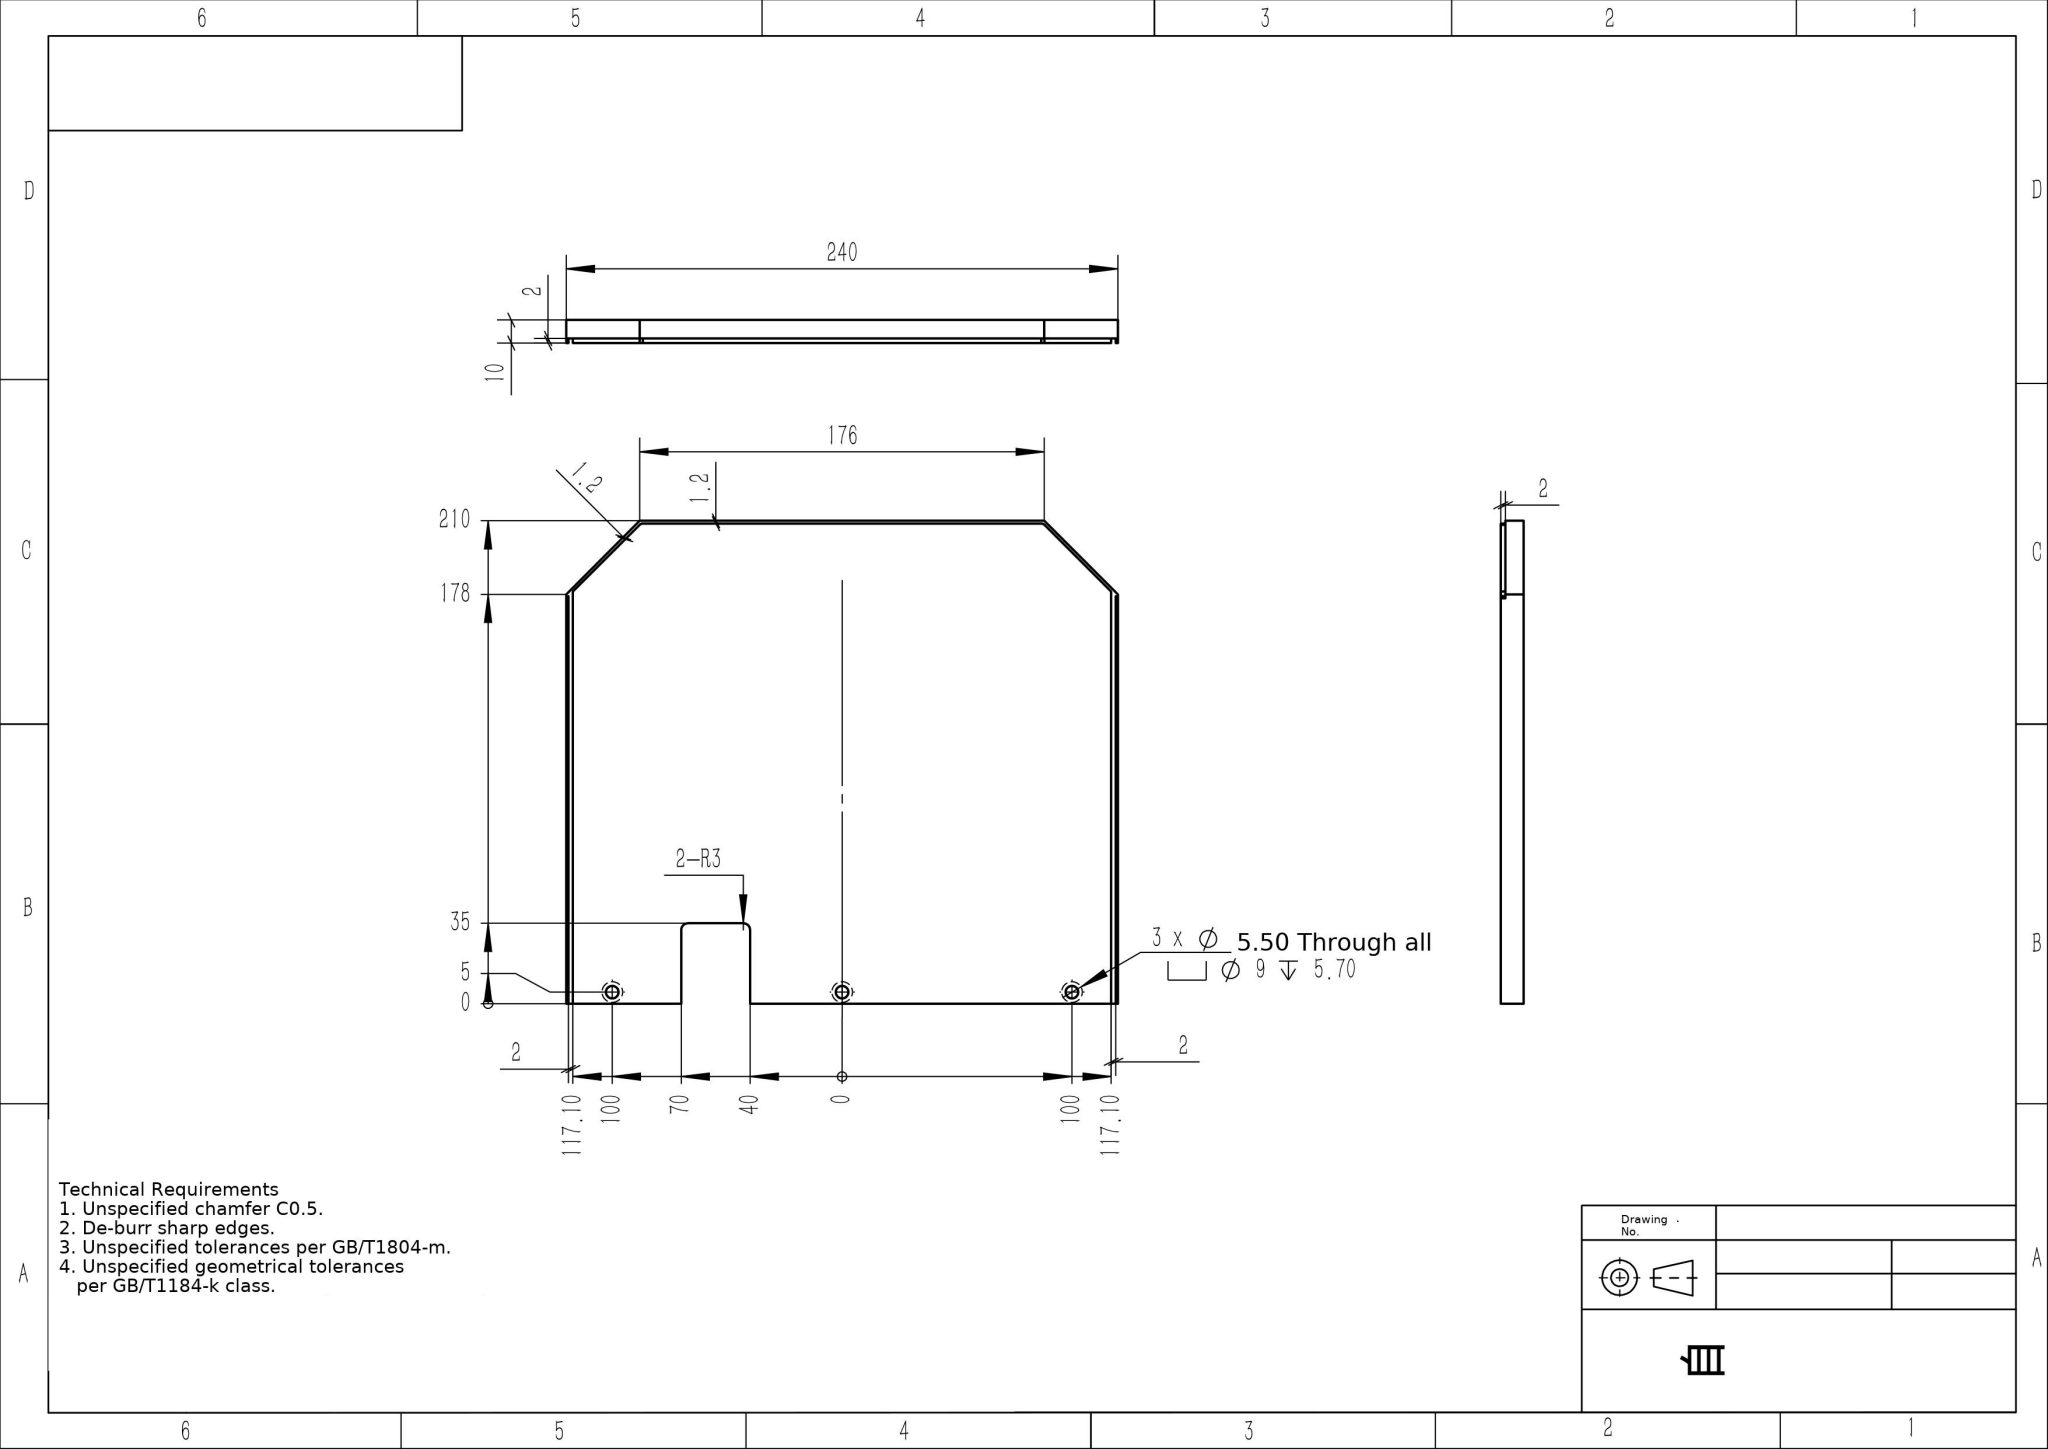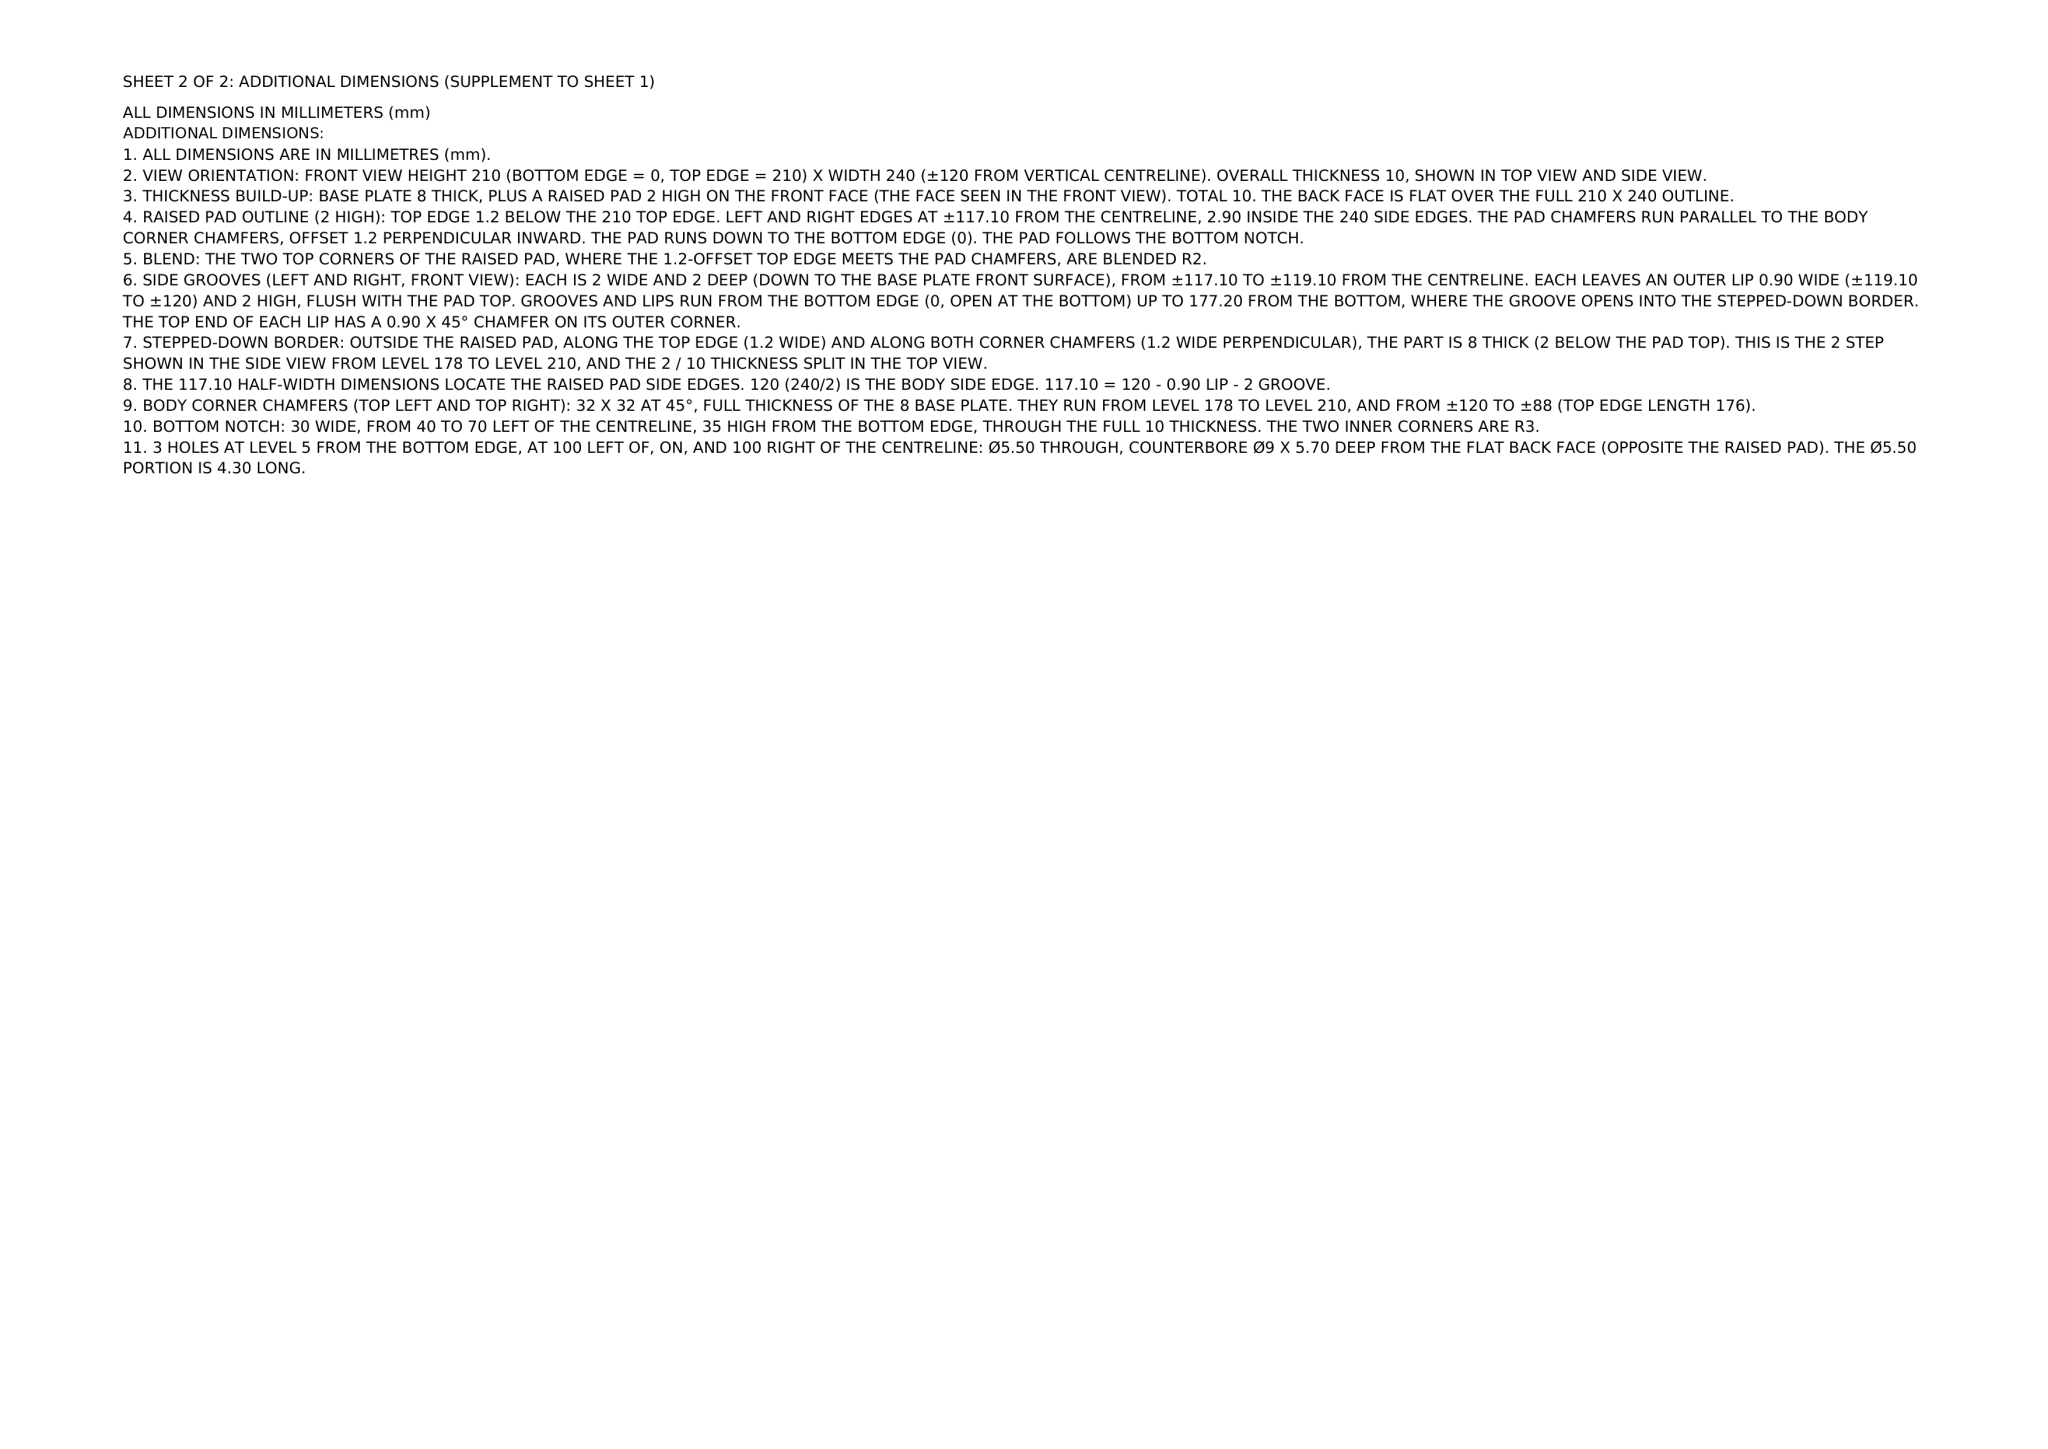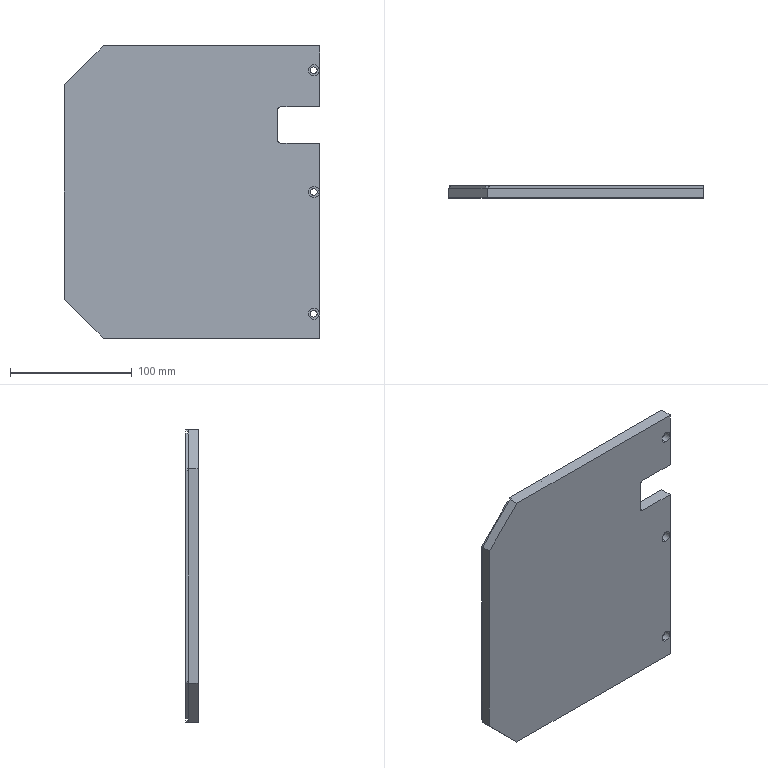Part | NX | mm | Chamfered Trapezoidal Mounting Panel | 1 solid | 43 faces | box 210 x 10 x 240 mm | volume 479838 mm3 | plane 27 | cylinder 16 | commonest cylinder face diameters 9 x6 5.5 x6 4 x2 6 x2